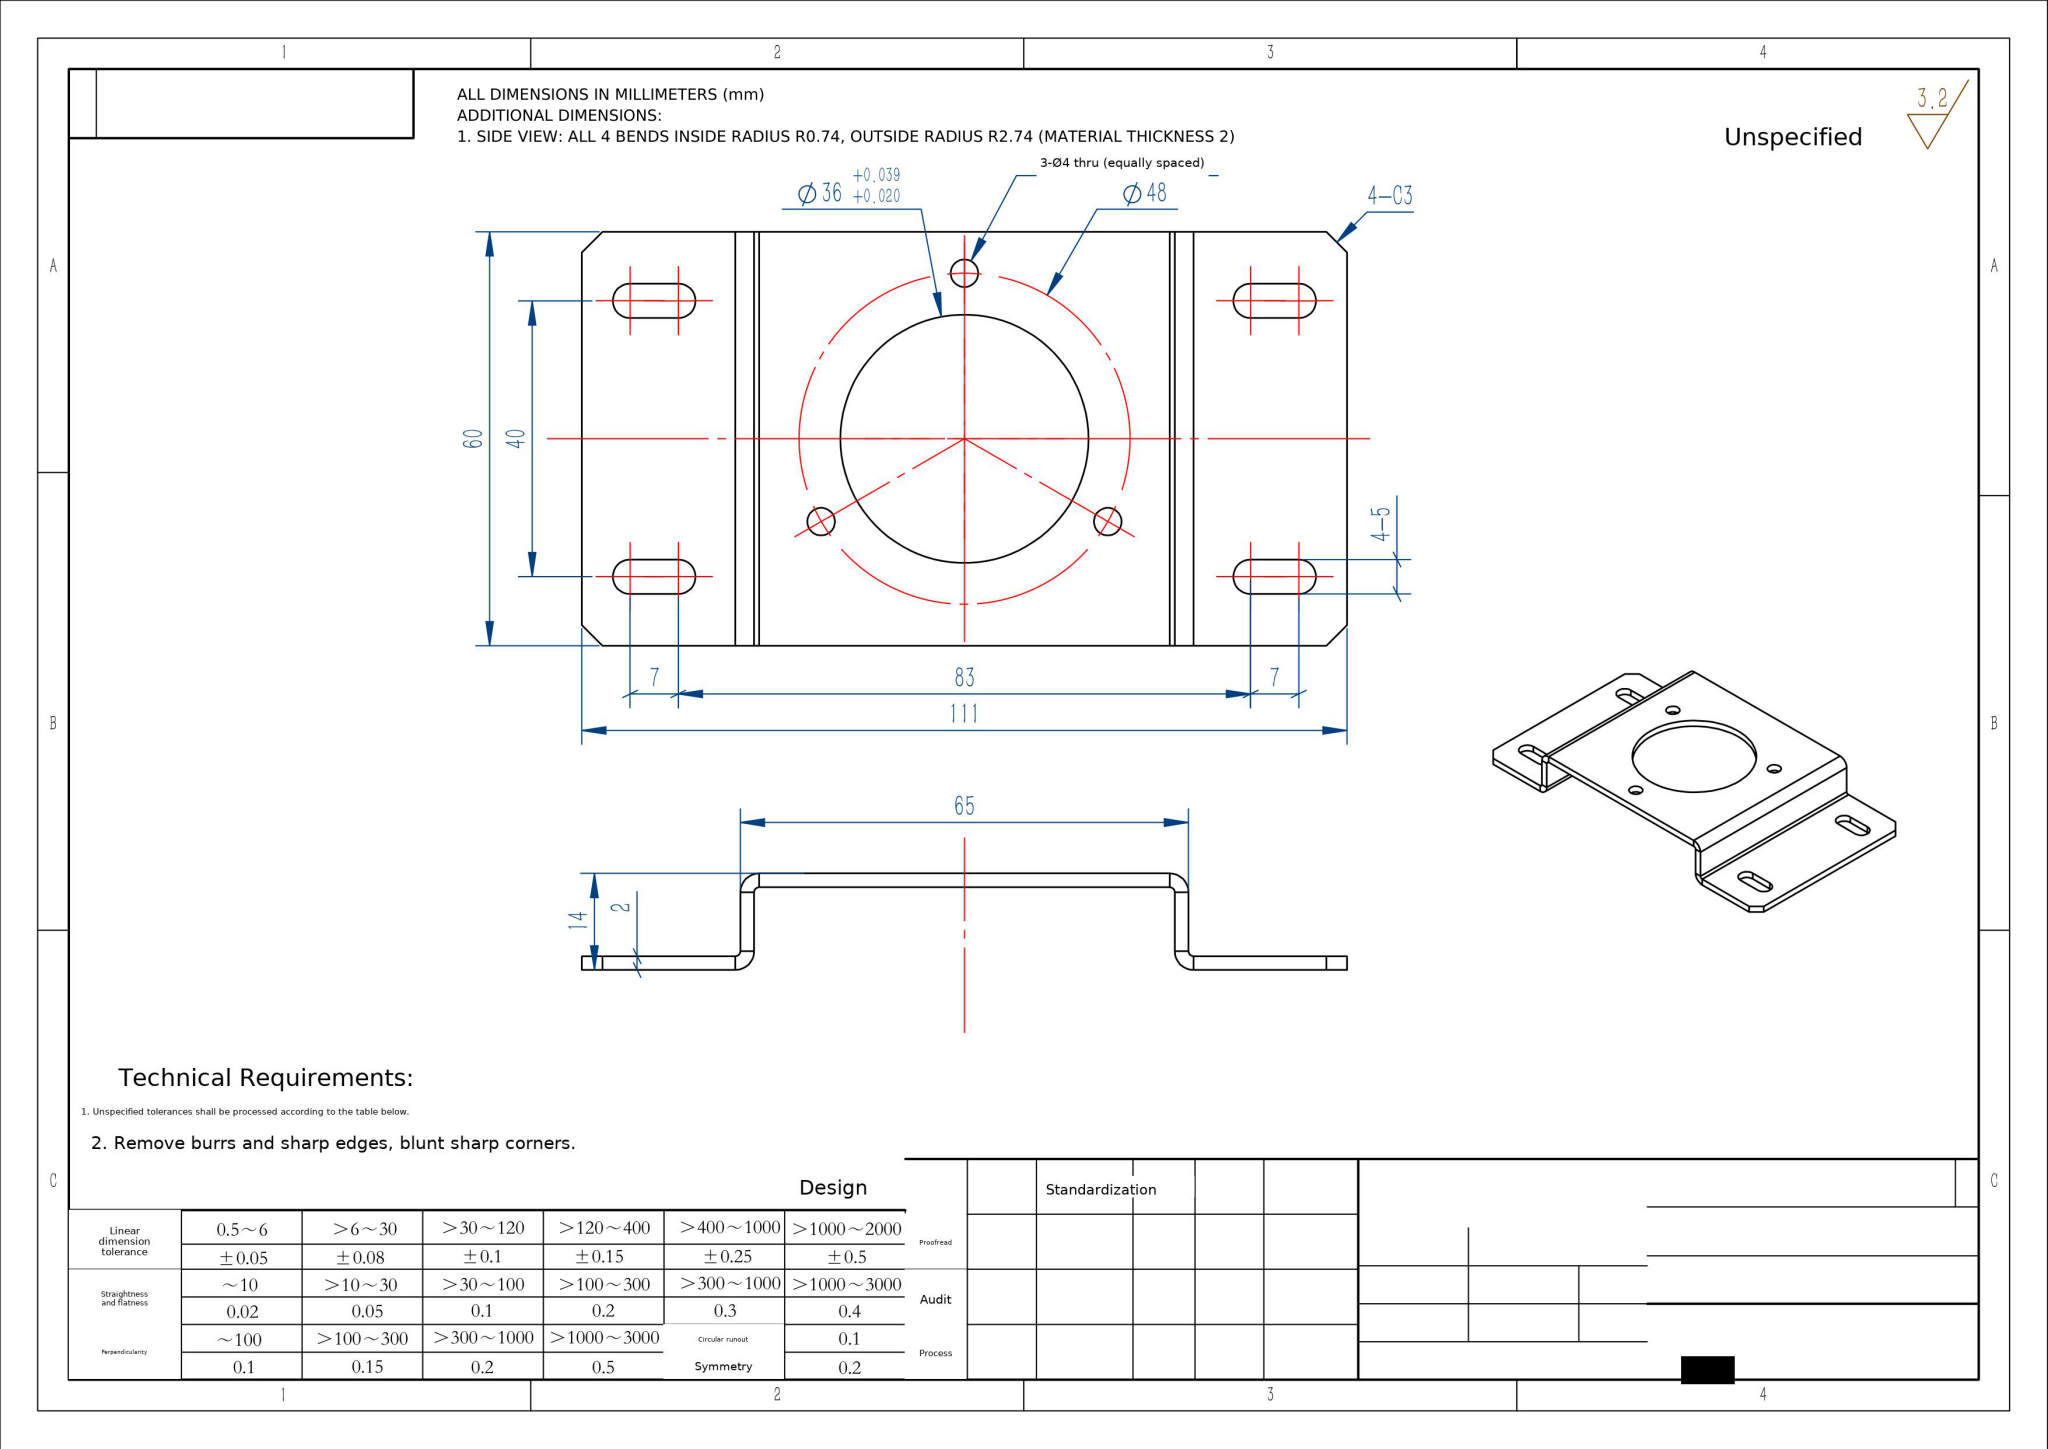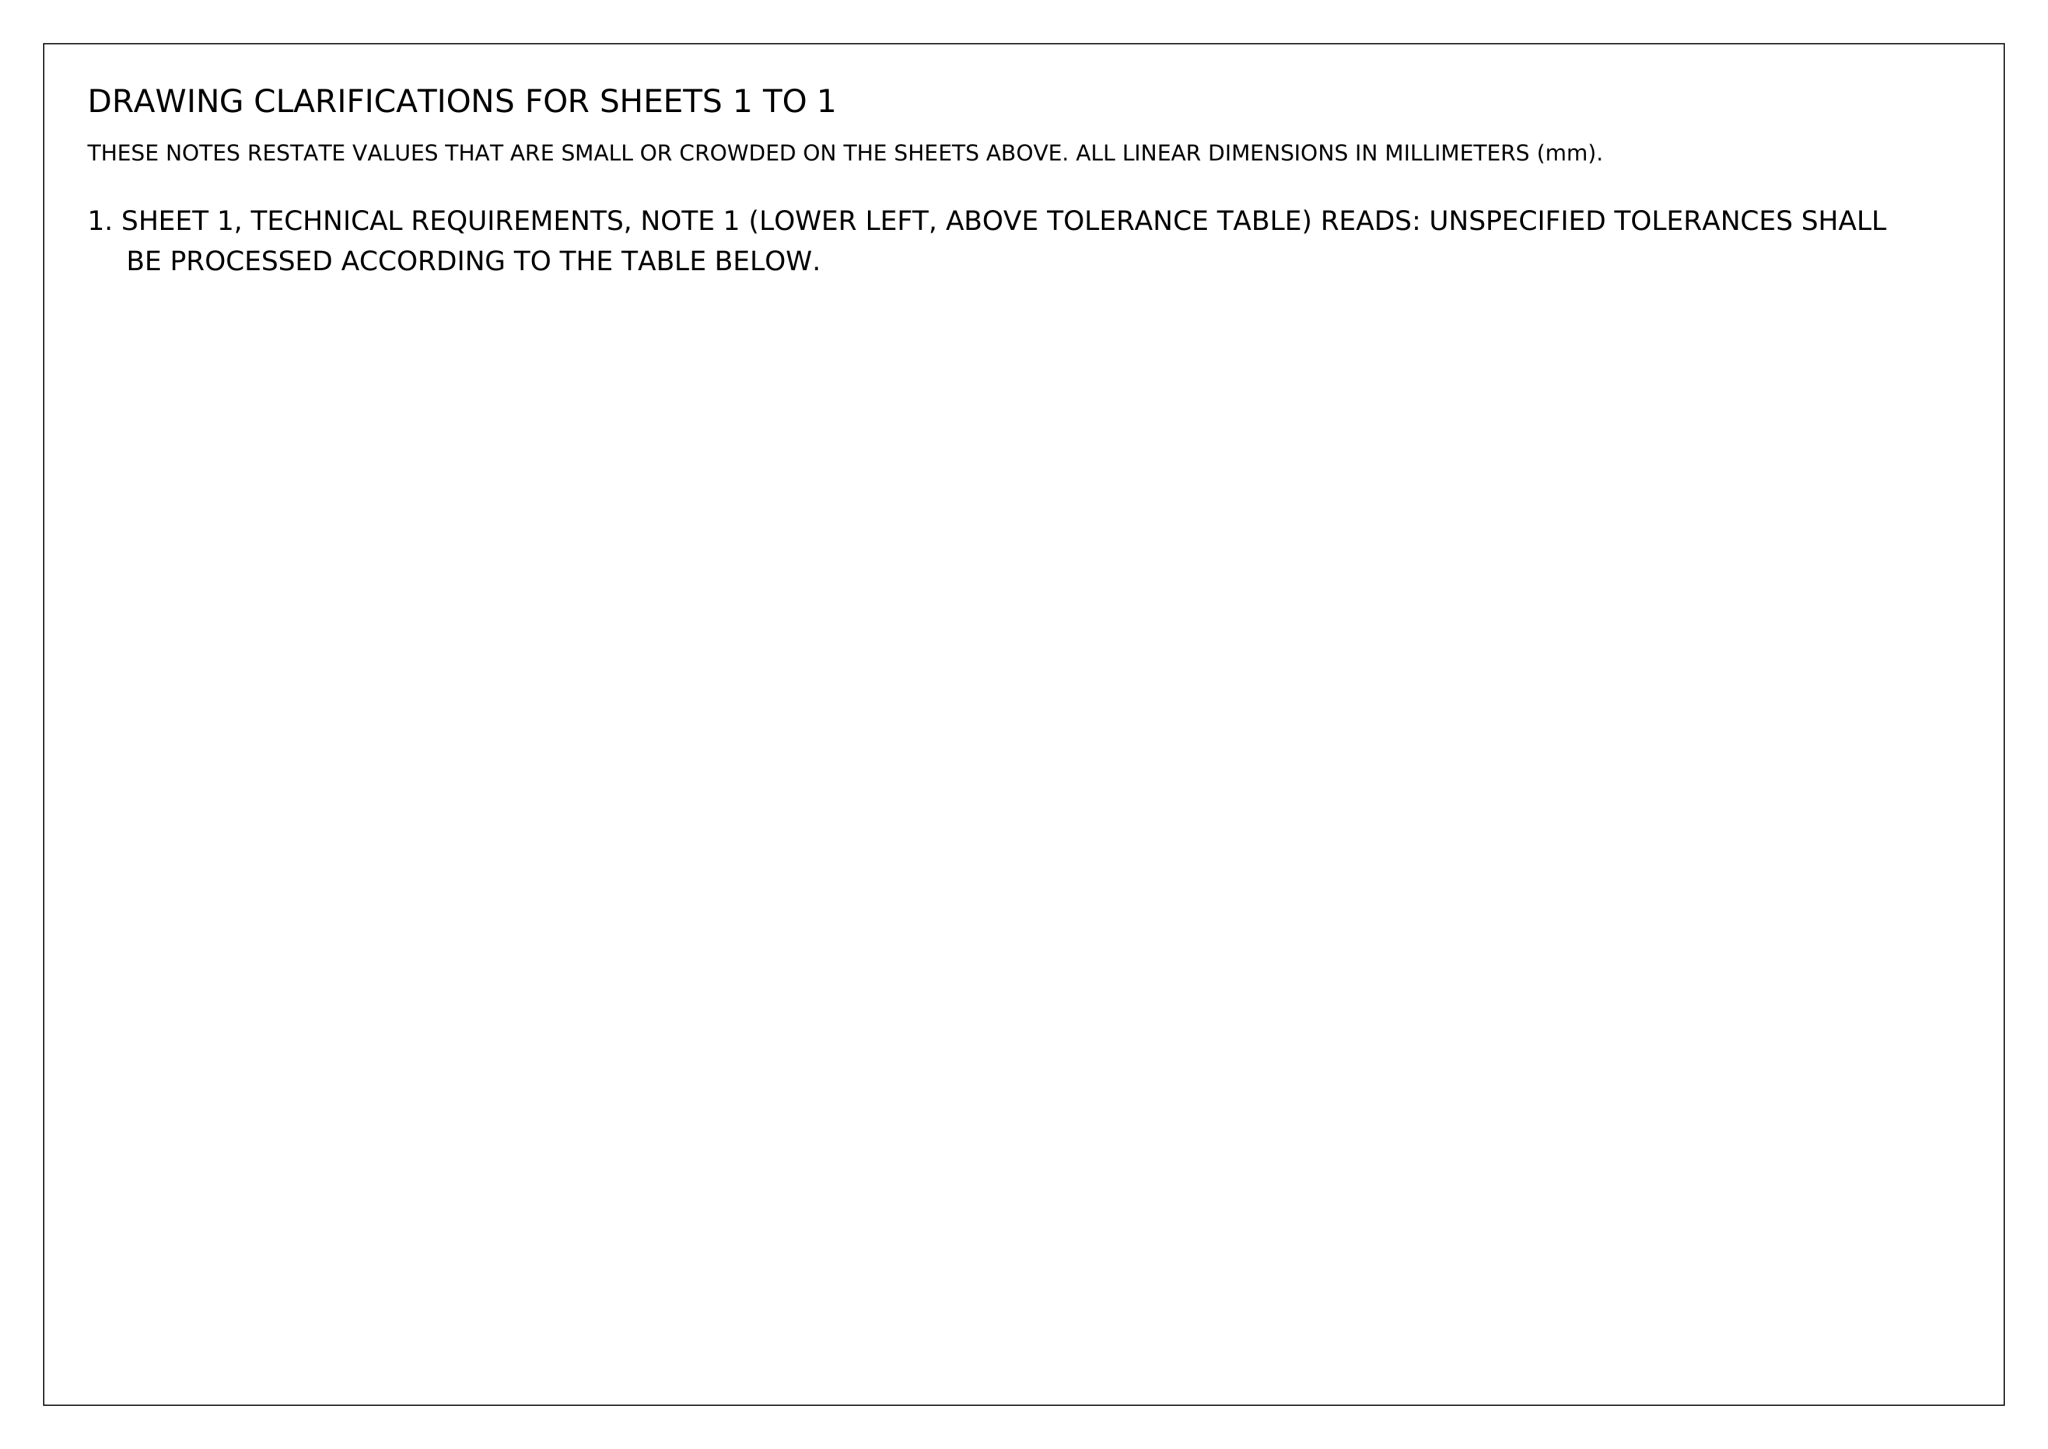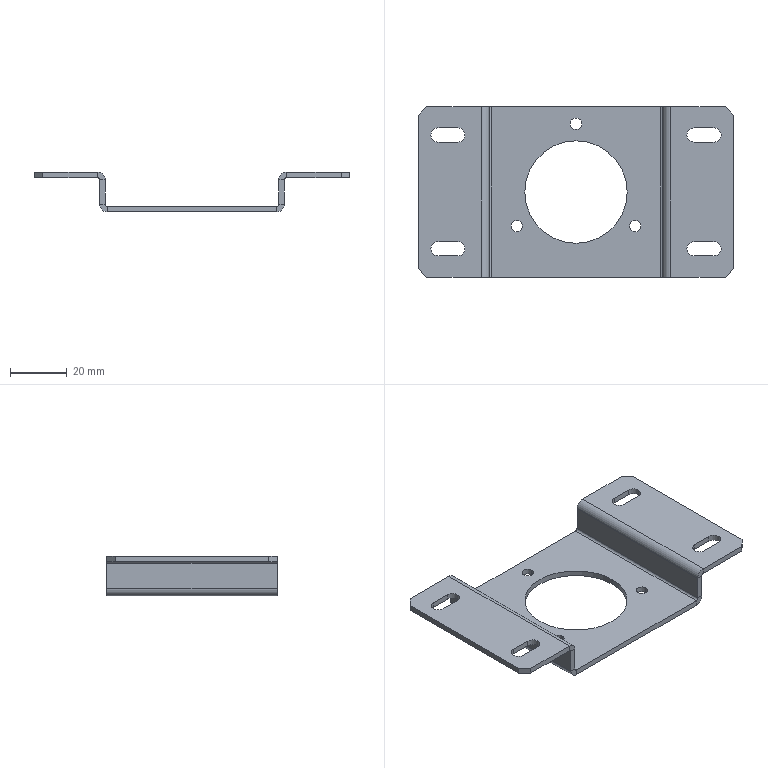Part | NX | mm | 1 solid | 70 faces | box 111 x 60 x 14 mm | volume 13258 mm3 | plane 42 | cylinder 28 | commonest cylinder face diameters 5 x12 4 x6 5.473 x4 1.473 x4 36 x2